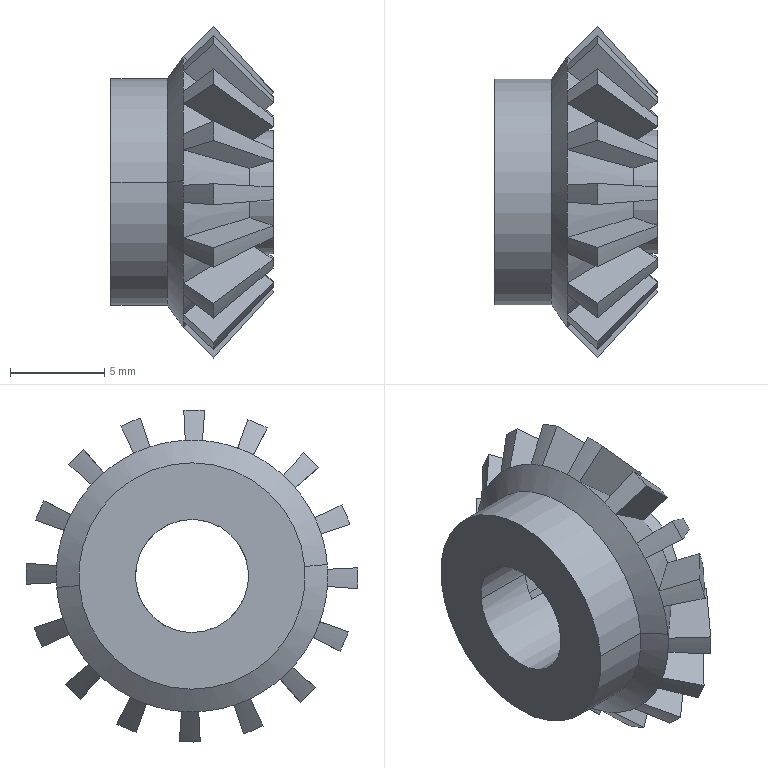Component | SolidWorks | X2_5851659952369525_X0_b_X2_7120_X0-3 | 1 solid | 111 faces | volume 728 mm3 | cone 66 | plane 39 | cylinder 6 | commonest cylinder face diameters 6.544 x2 12 x2 6 x2